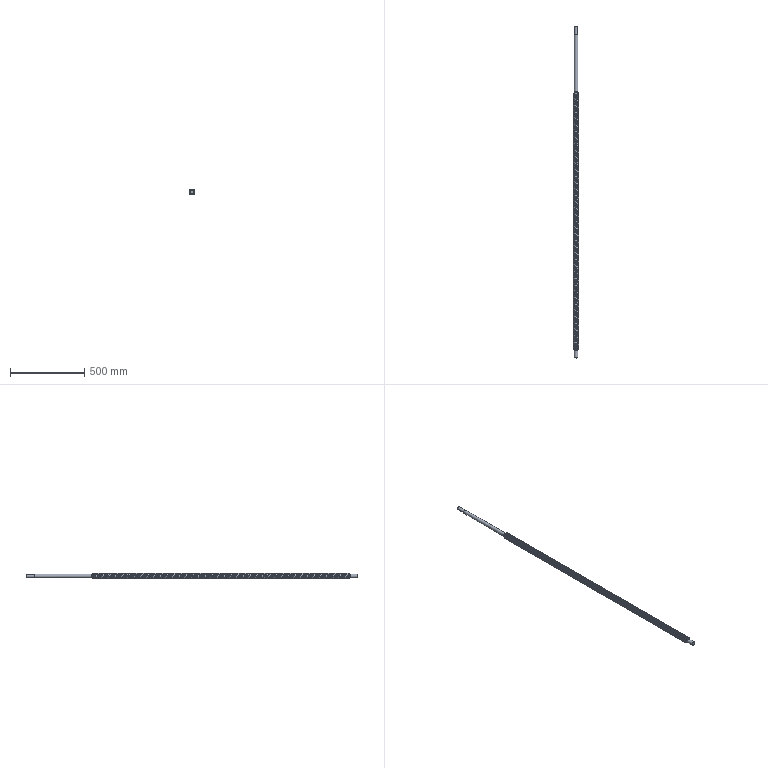Component | NX | LEAD_SCREW | 1 solid | 16 faces | volume 1883468 mm3 | plane 7 | cylinder 6 | spline 3 | commonest cylinder face diameters 25 x2 24 x2 40 x1 20 x1